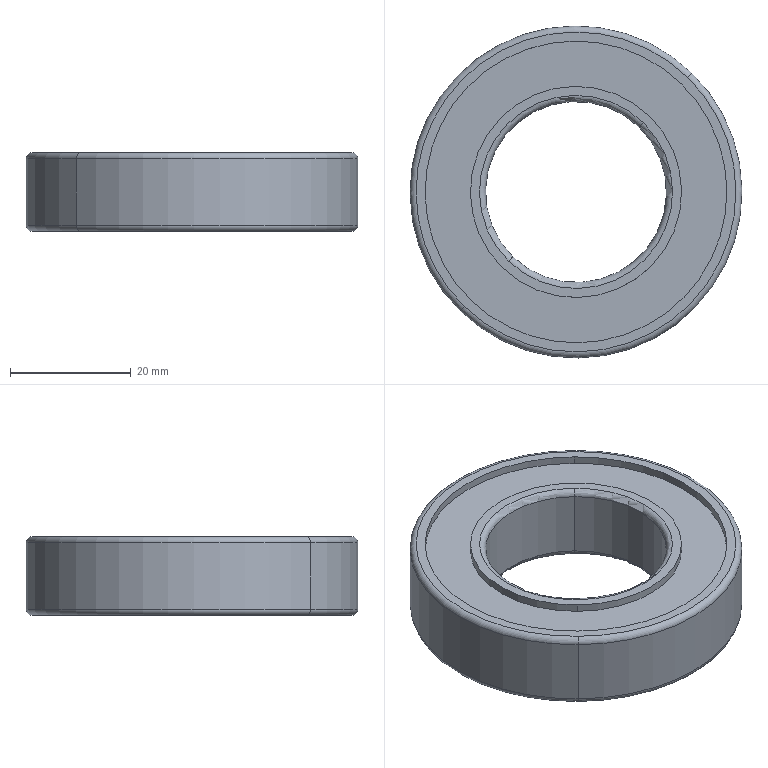Component | SolidWorks | 12AEncoderWheel-1_12A6006RZBearing-1 | 1 solid | 26 faces | box 55 x 55 x 13 mm | volume 18978 mm3 | cylinder 12 | torus 8 | plane 6 | commonest cylinder face diameters 50 x4 35 x4 55 x2 30 x2
STEP:
#1=CARTESIAN_POINT('',(5.515,6.57,0.2657));
#2=VERTEX_POINT('',#1);
#3=CARTESIAN_POINT('',(4.004,5.019,0.2657));
#4=VERTEX_POINT('',#3);
#5=CARTESIAN_POINT('',(4.76,5.795,0.2657));
#6=DIRECTION('',(0.,0.,1.));
#7=DIRECTION('',(-0.6982,-0.7159,0.));
#8=AXIS2_PLACEMENT_3D('',#5,#6,#7);
#9=CIRCLE('',#8,1.083);
#10=EDGE_CURVE('',#2,#4,#9,.T.);
#11=ORIENTED_EDGE('',*,*,#10,.F.);
#12=CARTESIAN_POINT('',(5.515,6.57,-0.1673));
#13=VERTEX_POINT('',#12);
#14=CARTESIAN_POINT('',(5.515,6.57,197.156));
#15=DIRECTION('',(-0.,-0.,-1.));
#16=VECTOR('',#15,39.37);
#17=LINE('',#14,#16);
#18=EDGE_CURVE('',#2,#13,#17,.T.);
#19=ORIENTED_EDGE('',*,*,#18,.T.);
#20=CARTESIAN_POINT('',(4.004,5.019,-0.1673));
#21=VERTEX_POINT('',#20);
#22=CARTESIAN_POINT('',(4.76,5.795,-0.1673));
#23=DIRECTION('',(0.,0.,1.));
#24=DIRECTION('',(-0.6982,-0.7159,0.));
#25=AXIS2_PLACEMENT_3D('',#22,#23,#24);
#26=CIRCLE('',#25,1.083);
#27=EDGE_CURVE('',#13,#21,#26,.T.);
#28=ORIENTED_EDGE('',*,*,#27,.T.);
#29=CARTESIAN_POINT('',(4.004,5.019,197.156));
#30=DIRECTION('',(-0.,-0.,-1.));
#31=VECTOR('',#30,39.37);
#32=LINE('',#29,#31);
#33=EDGE_CURVE('',#4,#21,#32,.T.);
#34=ORIENTED_EDGE('',*,*,#33,.F.);
#35=EDGE_LOOP('',(#11,#19,#28,#34));
#36=FACE_OUTER_BOUND('',#35,.T.);
#37=CARTESIAN_POINT('',(4.76,5.795,197.156));
#38=DIRECTION('',(-0.,-0.,-1.));
#39=DIRECTION('',(-0.6982,-0.7159,0.));
#40=AXIS2_PLACEMENT_3D('',#37,#38,#39);
#41=CYLINDRICAL_SURFACE('',#40,1.083);
#42=ADVANCED_FACE('',(#36),#41,.T.);
#43=CARTESIAN_POINT('',(4.76,5.795,0.2657));
#44=DIRECTION('',(0.,0.,1.));
#45=DIRECTION('',(-0.6982,-0.7159,0.));
#46=AXIS2_PLACEMENT_3D('',#43,#44,#45);
#47=CIRCLE('',#46,1.083);
#48=EDGE_CURVE('',#4,#2,#47,.T.);
#49=ORIENTED_EDGE('',*,*,#48,.T.);
#50=CARTESIAN_POINT('',(5.488,6.541,0.3051));
#51=VERTEX_POINT('',#50);
#52=CARTESIAN_POINT('',(5.488,6.541,0.2657));
#53=DIRECTION('',(0.7159,-0.6982,0.));
#54=DIRECTION('',(0.6982,0.7159,0.));
#55=AXIS2_PLACEMENT_3D('',#52,#53,#54);
#56=CIRCLE('',#55,0.03937);
#57=EDGE_CURVE('',#2,#51,#56,.T.);
#58=ORIENTED_EDGE('',*,*,#57,.T.);
#59=CARTESIAN_POINT('',(4.031,5.048,0.3051));
#60=VERTEX_POINT('',#59);
#61=CARTESIAN_POINT('',(4.76,5.795,0.3051));
#62=DIRECTION('',(0.,0.,1.));
#63=DIRECTION('',(-0.6982,-0.7159,0.));
#64=AXIS2_PLACEMENT_3D('',#61,#62,#63);
#65=CIRCLE('',#64,1.043);
#66=EDGE_CURVE('',#60,#51,#65,.T.);
#67=ORIENTED_EDGE('',*,*,#66,.F.);
#68=CARTESIAN_POINT('',(4.031,5.048,0.2657));
#69=DIRECTION('',(-0.7159,0.6982,-0.));
#70=DIRECTION('',(-0.6982,-0.7159,0.));
#71=AXIS2_PLACEMENT_3D('',#68,#69,#70);
#72=CIRCLE('',#71,0.03937);
#73=EDGE_CURVE('',#4,#60,#72,.T.);
#74=ORIENTED_EDGE('',*,*,#73,.F.);
#75=EDGE_LOOP('',(#49,#58,#67,#74));
#76=FACE_OUTER_BOUND('',#75,.T.);
#77=CARTESIAN_POINT('',(4.76,5.795,0.2657));
#78=DIRECTION('',(0.,0.,1.));
#79=DIRECTION('',(-0.6982,-0.7159,0.));
#80=AXIS2_PLACEMENT_3D('',#77,#78,#79);
#81=TOROIDAL_SURFACE('',#80,1.043,0.03937);
#82=ADVANCED_FACE('',(#76),#81,.T.);
#83=CARTESIAN_POINT('',(4.072,5.09,0.3051));
#84=VERTEX_POINT('',#83);
#85=CARTESIAN_POINT('',(5.447,6.499,0.3051));
#86=VERTEX_POINT('',#85);
#87=CARTESIAN_POINT('',(4.76,5.795,0.3051));
#88=DIRECTION('',(0.,0.,1.));
#89=DIRECTION('',(-0.6982,-0.7159,0.));
#90=AXIS2_PLACEMENT_3D('',#87,#88,#89);
#91=CIRCLE('',#90,0.9843);
#92=EDGE_CURVE('',#84,#86,#91,.T.);
#93=ORIENTED_EDGE('',*,*,#92,.T.);
#94=CARTESIAN_POINT('',(5.447,6.499,0.2539));
#95=VERTEX_POINT('',#94);
#96=CARTESIAN_POINT('',(5.447,6.499,197.156));
#97=DIRECTION('',(-0.,-0.,-1.));
#98=VECTOR('',#97,39.37);
#99=LINE('',#96,#98);
#100=EDGE_CURVE('',#86,#95,#99,.T.);
#101=ORIENTED_EDGE('',*,*,#100,.T.);
#102=CARTESIAN_POINT('',(4.072,5.09,0.2539));
#103=VERTEX_POINT('',#102);
#104=CARTESIAN_POINT('',(4.76,5.795,0.2539));
#105=DIRECTION('',(0.,0.,1.));
#106=DIRECTION('',(-0.6982,-0.7159,0.));
#107=AXIS2_PLACEMENT_3D('',#104,#105,#106);
#108=CIRCLE('',#107,0.9843);
#109=EDGE_CURVE('',#103,#95,#108,.T.);
#110=ORIENTED_EDGE('',*,*,#109,.F.);
#111=CARTESIAN_POINT('',(4.072,5.09,197.156));
#112=DIRECTION('',(-0.,-0.,-1.));
#113=VECTOR('',#112,39.37);
#114=LINE('',#111,#113);
#115=EDGE_CURVE('',#84,#103,#114,.T.);
#116=ORIENTED_EDGE('',*,*,#115,.F.);
#117=EDGE_LOOP('',(#93,#101,#110,#116));
#118=FACE_OUTER_BOUND('',#117,.T.);
#119=CARTESIAN_POINT('',(4.76,5.795,197.156));
#120=DIRECTION('',(-0.,-0.,-1.));
#121=DIRECTION('',(-0.6982,-0.7159,0.));
#122=AXIS2_PLACEMENT_3D('',#119,#120,#121);
#123=CYLINDRICAL_SURFACE('',#122,0.9843);
#124=ADVANCED_FACE('',(#118),#123,.F.);
#125=CARTESIAN_POINT('',(5.241,6.288,0.3051));
#126=VERTEX_POINT('',#125);
#127=CARTESIAN_POINT('',(4.279,5.301,0.3051));
#128=VERTEX_POINT('',#127);
#129=CARTESIAN_POINT('',(4.76,5.795,0.3051));
#130=DIRECTION('',(0.,0.,1.));
#131=DIRECTION('',(-0.6982,-0.7159,0.));
#132=AXIS2_PLACEMENT_3D('',#129,#130,#131);
#133=CIRCLE('',#132,0.689);
#134=EDGE_CURVE('',#126,#128,#133,.T.);
#135=ORIENTED_EDGE('',*,*,#134,.F.);
#136=CARTESIAN_POINT('',(5.241,6.288,0.2539));
#137=VERTEX_POINT('',#136);
#138=CARTESIAN_POINT('',(5.241,6.288,197.156));
#139=DIRECTION('',(-0.,-0.,-1.));
#140=VECTOR('',#139,39.37);
#141=LINE('',#138,#140);
#142=EDGE_CURVE('',#126,#137,#141,.T.);
#143=ORIENTED_EDGE('',*,*,#142,.T.);
#144=CARTESIAN_POINT('',(4.279,5.301,0.2539));
#145=VERTEX_POINT('',#144);
#146=CARTESIAN_POINT('',(4.76,5.795,0.2539));
#147=DIRECTION('',(0.,0.,1.));
#148=DIRECTION('',(-0.6982,-0.7159,0.));
#149=AXIS2_PLACEMENT_3D('',#146,#147,#148);
#150=CIRCLE('',#149,0.689);
#151=EDGE_CURVE('',#137,#145,#150,.T.);
#152=ORIENTED_EDGE('',*,*,#151,.T.);
#153=CARTESIAN_POINT('',(4.279,5.301,197.156));
#154=DIRECTION('',(-0.,-0.,-1.));
#155=VECTOR('',#154,39.37);
#156=LINE('',#153,#155);
#157=EDGE_CURVE('',#128,#145,#156,.T.);
#158=ORIENTED_EDGE('',*,*,#157,.F.);
#159=EDGE_LOOP('',(#135,#143,#152,#158));
#160=FACE_OUTER_BOUND('',#159,.T.);
#161=CARTESIAN_POINT('',(4.76,5.795,197.156));
#162=DIRECTION('',(-0.,-0.,-1.));
#163=DIRECTION('',(-0.6982,-0.7159,0.));
#164=AXIS2_PLACEMENT_3D('',#161,#162,#163);
#165=CYLINDRICAL_SURFACE('',#164,0.689);
#166=ADVANCED_FACE('',(#160),#165,.T.);
#167=CARTESIAN_POINT('',(4.32,5.344,0.3051));
#168=VERTEX_POINT('',#167);
#169=CARTESIAN_POINT('',(5.199,6.246,0.3051));
#170=VERTEX_POINT('',#169);
#171=CARTESIAN_POINT('',(4.76,5.795,0.3051));
#172=DIRECTION('',(0.,0.,1.));
#173=DIRECTION('',(-0.6982,-0.7159,0.));
#174=AXIS2_PLACEMENT_3D('',#171,#172,#173);
#175=CIRCLE('',#174,0.6299);
#176=EDGE_CURVE('',#168,#170,#175,.T.);
#177=ORIENTED_EDGE('',*,*,#176,.T.);
#178=CARTESIAN_POINT('',(5.172,6.217,0.2657));
#179=VERTEX_POINT('',#178);
#180=CARTESIAN_POINT('',(5.199,6.246,0.2657));
#181=DIRECTION('',(0.7159,-0.6982,0.));
#182=DIRECTION('',(0.6982,0.7159,0.));
#183=AXIS2_PLACEMENT_3D('',#180,#181,#182);
#184=CIRCLE('',#183,0.03937);
#185=EDGE_CURVE('',#170,#179,#184,.T.);
#186=ORIENTED_EDGE('',*,*,#185,.T.);
#187=CARTESIAN_POINT('',(4.347,5.372,0.2657));
#188=VERTEX_POINT('',#187);
#189=CARTESIAN_POINT('',(4.76,5.795,0.2657));
#190=DIRECTION('',(0.,0.,1.));
#191=DIRECTION('',(-0.6982,-0.7159,0.));
#192=AXIS2_PLACEMENT_3D('',#189,#190,#191);
#193=CIRCLE('',#192,0.5906);
#194=EDGE_CURVE('',#188,#179,#193,.T.);
#195=ORIENTED_EDGE('',*,*,#194,.F.);
#196=CARTESIAN_POINT('',(4.32,5.344,0.2657));
#197=DIRECTION('',(-0.7159,0.6982,-0.));
#198=DIRECTION('',(-0.6982,-0.7159,0.));
#199=AXIS2_PLACEMENT_3D('',#196,#197,#198);
#200=CIRCLE('',#199,0.03937);
#201=EDGE_CURVE('',#168,#188,#200,.T.);
#202=ORIENTED_EDGE('',*,*,#201,.F.);
#203=EDGE_LOOP('',(#177,#186,#195,#202));
#204=FACE_OUTER_BOUND('',#203,.T.);
#205=CARTESIAN_POINT('',(4.76,5.795,0.2657));
#206=DIRECTION('',(0.,0.,1.));
#207=DIRECTION('',(-0.6982,-0.7159,0.));
#208=AXIS2_PLACEMENT_3D('',#205,#206,#207);
#209=TOROIDAL_SURFACE('',#208,0.6299,0.03937);
#210=ADVANCED_FACE('',(#204),#209,.T.);
#211=ORIENTED_EDGE('',*,*,#194,.T.);
#212=CARTESIAN_POINT('',(5.172,6.217,-0.1673));
#213=VERTEX_POINT('',#212);
#214=CARTESIAN_POINT('',(5.172,6.217,197.156));
#215=DIRECTION('',(-0.,-0.,-1.));
#216=VECTOR('',#215,39.37);
#217=LINE('',#214,#216);
#218=EDGE_CURVE('',#179,#213,#217,.T.);
#219=ORIENTED_EDGE('',*,*,#218,.T.);
#220=CARTESIAN_POINT('',(4.347,5.372,-0.1673));
#221=VERTEX_POINT('',#220);
#222=CARTESIAN_POINT('',(4.76,5.795,-0.1673));
#223=DIRECTION('',(0.,0.,1.));
#224=DIRECTION('',(-0.6982,-0.7159,0.));
#225=AXIS2_PLACEMENT_3D('',#222,#223,#224);
#226=CIRCLE('',#225,0.5906);
#227=EDGE_CURVE('',#221,#213,#226,.T.);
#228=ORIENTED_EDGE('',*,*,#227,.F.);
#229=CARTESIAN_POINT('',(4.347,5.372,197.156));
#230=DIRECTION('',(-0.,-0.,-1.));
#231=VECTOR('',#230,39.37);
#232=LINE('',#229,#231);
#233=EDGE_CURVE('',#188,#221,#232,.T.);
#234=ORIENTED_EDGE('',*,*,#233,.F.);
#235=EDGE_LOOP('',(#211,#219,#228,#234));
#236=FACE_OUTER_BOUND('',#235,.T.);
#237=CARTESIAN_POINT('',(4.76,5.795,197.156));
#238=DIRECTION('',(-0.,-0.,-1.));
#239=DIRECTION('',(-0.6982,-0.7159,0.));
#240=AXIS2_PLACEMENT_3D('',#237,#238,#239);
#241=CYLINDRICAL_SURFACE('',#240,0.5906);
#242=ADVANCED_FACE('',(#236),#241,.F.);
#243=ORIENTED_EDGE('',*,*,#227,.T.);
#244=CARTESIAN_POINT('',(5.199,6.246,-0.2067));
#245=VERTEX_POINT('',#244);
#246=CARTESIAN_POINT('',(5.199,6.246,-0.1673));
#247=DIRECTION('',(0.7159,-0.6982,0.));
#248=DIRECTION('',(0.6982,0.7159,0.));
#249=AXIS2_PLACEMENT_3D('',#246,#247,#248);
#250=CIRCLE('',#249,0.03937);
#251=EDGE_CURVE('',#213,#245,#250,.T.);
#252=ORIENTED_EDGE('',*,*,#251,.T.);
#253=CARTESIAN_POINT('',(4.32,5.344,-0.2067));
#254=VERTEX_POINT('',#253);
#255=CARTESIAN_POINT('',(4.76,5.795,-0.2067));
#256=DIRECTION('',(0.,0.,1.));
#257=DIRECTION('',(-0.6982,-0.7159,0.));
#258=AXIS2_PLACEMENT_3D('',#255,#256,#257);
#259=CIRCLE('',#258,0.6299);
#260=EDGE_CURVE('',#254,#245,#259,.T.);
#261=ORIENTED_EDGE('',*,*,#260,.F.);
#262=CARTESIAN_POINT('',(4.32,5.344,-0.1673));
#263=DIRECTION('',(-0.7159,0.6982,-0.));
#264=DIRECTION('',(-0.6982,-0.7159,0.));
#265=AXIS2_PLACEMENT_3D('',#262,#263,#264);
#266=CIRCLE('',#265,0.03937);
#267=EDGE_CURVE('',#221,#254,#266,.T.);
#268=ORIENTED_EDGE('',*,*,#267,.F.);
#269=EDGE_LOOP('',(#243,#252,#261,#268));
#270=FACE_OUTER_BOUND('',#269,.T.);
#271=CARTESIAN_POINT('',(4.76,5.795,-0.1673));
#272=DIRECTION('',(0.,0.,1.));
#273=DIRECTION('',(-0.6982,-0.7159,0.));
#274=AXIS2_PLACEMENT_3D('',#271,#272,#273);
#275=TOROIDAL_SURFACE('',#274,0.6299,0.03937);
#276=ADVANCED_FACE('',(#270),#275,.T.);
#277=CARTESIAN_POINT('',(5.241,6.288,-0.1555));
#278=VERTEX_POINT('',#277);
#279=CARTESIAN_POINT('',(4.279,5.301,-0.1555));
#280=VERTEX_POINT('',#279);
#281=CARTESIAN_POINT('',(4.76,5.795,-0.1555));
#282=DIRECTION('',(0.,0.,1.));
#283=DIRECTION('',(-0.6982,-0.7159,0.));
#284=AXIS2_PLACEMENT_3D('',#281,#282,#283);
#285=CIRCLE('',#284,0.689);
#286=EDGE_CURVE('',#278,#280,#285,.T.);
#287=ORIENTED_EDGE('',*,*,#286,.F.);
#288=CARTESIAN_POINT('',(5.241,6.288,-0.2067));
#289=VERTEX_POINT('',#288);
#290=CARTESIAN_POINT('',(5.241,6.288,197.156));
#291=DIRECTION('',(-0.,-0.,-1.));
#292=VECTOR('',#291,39.37);
#293=LINE('',#290,#292);
#294=EDGE_CURVE('',#278,#289,#293,.T.);
#295=ORIENTED_EDGE('',*,*,#294,.T.);
#296=CARTESIAN_POINT('',(4.279,5.301,-0.2067));
#297=VERTEX_POINT('',#296);
#298=CARTESIAN_POINT('',(4.76,5.795,-0.2067));
#299=DIRECTION('',(0.,0.,1.));
#300=DIRECTION('',(-0.6982,-0.7159,0.));
#301=AXIS2_PLACEMENT_3D('',#298,#299,#300);
#302=CIRCLE('',#301,0.689);
#303=EDGE_CURVE('',#289,#297,#302,.T.);
#304=ORIENTED_EDGE('',*,*,#303,.T.);
#305=CARTESIAN_POINT('',(4.279,5.301,197.156));
#306=DIRECTION('',(-0.,-0.,-1.));
#307=VECTOR('',#306,39.37);
#308=LINE('',#305,#307);
#309=EDGE_CURVE('',#280,#297,#308,.T.);
#310=ORIENTED_EDGE('',*,*,#309,.F.);
#311=EDGE_LOOP('',(#287,#295,#304,#310));
#312=FACE_OUTER_BOUND('',#311,.T.);
#313=CARTESIAN_POINT('',(4.76,5.795,197.156));
#314=DIRECTION('',(-0.,-0.,-1.));
#315=DIRECTION('',(-0.6982,-0.7159,0.));
#316=AXIS2_PLACEMENT_3D('',#313,#314,#315);
#317=CYLINDRICAL_SURFACE('',#316,0.689);
#318=ADVANCED_FACE('',(#312),#317,.T.);
#319=CARTESIAN_POINT('',(4.072,5.09,-0.1555));
#320=VERTEX_POINT('',#319);
#321=CARTESIAN_POINT('',(5.447,6.499,-0.1555));
#322=VERTEX_POINT('',#321);
#323=CARTESIAN_POINT('',(4.76,5.795,-0.1555));
#324=DIRECTION('',(0.,0.,1.));
#325=DIRECTION('',(-0.6982,-0.7159,0.));
#326=AXIS2_PLACEMENT_3D('',#323,#324,#325);
#327=CIRCLE('',#326,0.9843);
#328=EDGE_CURVE('',#320,#322,#327,.T.);
#329=ORIENTED_EDGE('',*,*,#328,.T.);
#330=CARTESIAN_POINT('',(5.447,6.499,-0.2067));
#331=VERTEX_POINT('',#330);
#332=CARTESIAN_POINT('',(5.447,6.499,197.156));
#333=DIRECTION('',(-0.,-0.,-1.));
#334=VECTOR('',#333,39.37);
#335=LINE('',#332,#334);
#336=EDGE_CURVE('',#322,#331,#335,.T.);
#337=ORIENTED_EDGE('',*,*,#336,.T.);
#338=CARTESIAN_POINT('',(4.072,5.09,-0.2067));
#339=VERTEX_POINT('',#338);
#340=CARTESIAN_POINT('',(4.76,5.795,-0.2067));
#341=DIRECTION('',(0.,0.,1.));
#342=DIRECTION('',(-0.6982,-0.7159,0.));
#343=AXIS2_PLACEMENT_3D('',#340,#341,#342);
#344=CIRCLE('',#343,0.9843);
#345=EDGE_CURVE('',#339,#331,#344,.T.);
#346=ORIENTED_EDGE('',*,*,#345,.F.);
#347=CARTESIAN_POINT('',(4.072,5.09,197.156));
#348=DIRECTION('',(-0.,-0.,-1.));
#349=VECTOR('',#348,39.37);
#350=LINE('',#347,#349);
#351=EDGE_CURVE('',#320,#339,#350,.T.);
#352=ORIENTED_EDGE('',*,*,#351,.F.);
#353=EDGE_LOOP('',(#329,#337,#346,#352));
#354=FACE_OUTER_BOUND('',#353,.T.);
#355=CARTESIAN_POINT('',(4.76,5.795,197.156));
#356=DIRECTION('',(-0.,-0.,-1.));
#357=DIRECTION('',(-0.6982,-0.7159,0.));
#358=AXIS2_PLACEMENT_3D('',#355,#356,#357);
#359=CYLINDRICAL_SURFACE('',#358,0.9843);
#360=ADVANCED_FACE('',(#354),#359,.F.);
#361=CARTESIAN_POINT('',(4.031,5.048,-0.2067));
#362=VERTEX_POINT('',#361);
#363=CARTESIAN_POINT('',(5.488,6.541,-0.2067));
#364=VERTEX_POINT('',#363);
#365=CARTESIAN_POINT('',(4.76,5.795,-0.2067));
#366=DIRECTION('',(0.,0.,1.));
#367=DIRECTION('',(-0.6982,-0.7159,0.));
#368=AXIS2_PLACEMENT_3D('',#365,#366,#367);
#369=CIRCLE('',#368,1.043);
#370=EDGE_CURVE('',#362,#364,#369,.T.);
#371=ORIENTED_EDGE('',*,*,#370,.T.);
#372=CARTESIAN_POINT('',(5.488,6.541,-0.1673));
#373=DIRECTION('',(0.7159,-0.6982,0.));
#374=DIRECTION('',(0.6982,0.7159,0.));
#375=AXIS2_PLACEMENT_3D('',#372,#373,#374);
#376=CIRCLE('',#375,0.03937);
#377=EDGE_CURVE('',#364,#13,#376,.T.);
#378=ORIENTED_EDGE('',*,*,#377,.T.);
#379=CARTESIAN_POINT('',(4.76,5.795,-0.1673));
#380=DIRECTION('',(0.,0.,1.));
#381=DIRECTION('',(-0.6982,-0.7159,0.));
#382=AXIS2_PLACEMENT_3D('',#379,#380,#381);
#383=CIRCLE('',#382,1.083);
#384=EDGE_CURVE('',#21,#13,#383,.T.);
#385=ORIENTED_EDGE('',*,*,#384,.F.);
#386=CARTESIAN_POINT('',(4.031,5.048,-0.1673));
#387=DIRECTION('',(-0.7159,0.6982,-0.));
#388=DIRECTION('',(-0.6982,-0.7159,0.));
#389=AXIS2_PLACEMENT_3D('',#386,#387,#388);
#390=CIRCLE('',#389,0.03937);
#391=EDGE_CURVE('',#362,#21,#390,.T.);
#392=ORIENTED_EDGE('',*,*,#391,.F.);
#393=EDGE_LOOP('',(#371,#378,#385,#392));
#394=FACE_OUTER_BOUND('',#393,.T.);
#395=CARTESIAN_POINT('',(4.76,5.795,-0.1673));
#396=DIRECTION('',(0.,0.,1.));
#397=DIRECTION('',(-0.6982,-0.7159,0.));
#398=AXIS2_PLACEMENT_3D('',#395,#396,#397);
#399=TOROIDAL_SURFACE('',#398,1.043,0.03937);
#400=ADVANCED_FACE('',(#394),#399,.T.);
#401=ORIENTED_EDGE('',*,*,#377,.F.);
#402=CARTESIAN_POINT('',(4.76,5.795,-0.2067));
#403=DIRECTION('',(0.,0.,1.));
#404=DIRECTION('',(-0.6982,-0.7159,0.));
#405=AXIS2_PLACEMENT_3D('',#402,#403,#404);
#406=CIRCLE('',#405,1.043);
#407=EDGE_CURVE('',#364,#362,#406,.T.);
#408=ORIENTED_EDGE('',*,*,#407,.T.);
#409=ORIENTED_EDGE('',*,*,#391,.T.);
#410=ORIENTED_EDGE('',*,*,#27,.F.);
#411=EDGE_LOOP('',(#401,#408,#409,#410));
#412=FACE_OUTER_BOUND('',#411,.T.);
#413=CARTESIAN_POINT('',(4.76,5.795,-0.1673));
#414=DIRECTION('',(0.,0.,1.));
#415=DIRECTION('',(-0.6982,-0.7159,0.));
#416=AXIS2_PLACEMENT_3D('',#413,#414,#415);
#417=TOROIDAL_SURFACE('',#416,1.043,0.03937);
#418=ADVANCED_FACE('',(#412),#417,.T.);
#419=ORIENTED_EDGE('',*,*,#370,.F.);
#420=ORIENTED_EDGE('',*,*,#407,.F.);
#421=EDGE_LOOP('',(#419,#420));
#422=FACE_OUTER_BOUND('',#421,.T.);
#423=ORIENTED_EDGE('',*,*,#345,.T.);
#424=CARTESIAN_POINT('',(4.76,5.795,-0.2067));
#425=DIRECTION('',(0.,0.,1.));
#426=DIRECTION('',(-0.6982,-0.7159,0.));
#427=AXIS2_PLACEMENT_3D('',#424,#425,#426);
#428=CIRCLE('',#427,0.9843);
#429=EDGE_CURVE('',#331,#339,#428,.T.);
#430=ORIENTED_EDGE('',*,*,#429,.T.);
#431=EDGE_LOOP('',(#423,#430));
#432=FACE_BOUND('',#431,.T.);
#433=CARTESIAN_POINT('',(5.507,5.066,-0.2067));
#434=DIRECTION('',(-0.,-0.,-1.));
#435=DIRECTION('',(0.6982,0.7159,-0.));
#436=AXIS2_PLACEMENT_3D('',#433,#434,#435);
#437=PLANE('',#436);
#438=ADVANCED_FACE('',(#422,#432),#437,.T.);
#439=ORIENTED_EDGE('',*,*,#336,.F.);
#440=CARTESIAN_POINT('',(4.76,5.795,-0.1555));
#441=DIRECTION('',(0.,0.,1.));
#442=DIRECTION('',(-0.6982,-0.7159,0.));
#443=AXIS2_PLACEMENT_3D('',#440,#441,#442);
#444=CIRCLE('',#443,0.9843);
#445=EDGE_CURVE('',#322,#320,#444,.T.);
#446=ORIENTED_EDGE('',*,*,#445,.T.);
#447=ORIENTED_EDGE('',*,*,#351,.T.);
#448=ORIENTED_EDGE('',*,*,#429,.F.);
#449=EDGE_LOOP('',(#439,#446,#447,#448));
#450=FACE_OUTER_BOUND('',#449,.T.);
#451=CARTESIAN_POINT('',(4.76,5.795,197.156));
#452=DIRECTION('',(-0.,-0.,-1.));
#453=DIRECTION('',(-0.6982,-0.7159,0.));
#454=AXIS2_PLACEMENT_3D('',#451,#452,#453);
#455=CYLINDRICAL_SURFACE('',#454,0.9843);
#456=ADVANCED_FACE('',(#450),#455,.F.);
#457=ORIENTED_EDGE('',*,*,#328,.F.);
#458=ORIENTED_EDGE('',*,*,#445,.F.);
#459=EDGE_LOOP('',(#457,#458));
#460=FACE_OUTER_BOUND('',#459,.T.);
#461=CARTESIAN_POINT('',(4.76,5.795,-0.1555));
#462=DIRECTION('',(0.,0.,1.));
#463=DIRECTION('',(-0.6982,-0.7159,0.));
#464=AXIS2_PLACEMENT_3D('',#461,#462,#463);
#465=CIRCLE('',#464,0.689);
#466=EDGE_CURVE('',#280,#278,#465,.T.);
#467=ORIENTED_EDGE('',*,*,#466,.T.);
#468=ORIENTED_EDGE('',*,*,#286,.T.);
#469=EDGE_LOOP('',(#467,#468));
#470=FACE_BOUND('',#469,.T.);
#471=CARTESIAN_POINT('',(5.464,5.107,-0.1555));
#472=DIRECTION('',(-0.,-0.,-1.));
#473=DIRECTION('',(0.6982,0.7159,-0.));
#474=AXIS2_PLACEMENT_3D('',#471,#472,#473);
#475=PLANE('',#474);
#476=ADVANCED_FACE('',(#460,#470),#475,.T.);
#477=ORIENTED_EDGE('',*,*,#294,.F.);
#478=ORIENTED_EDGE('',*,*,#466,.F.);
#479=ORIENTED_EDGE('',*,*,#309,.T.);
#480=CARTESIAN_POINT('',(4.76,5.795,-0.2067));
#481=DIRECTION('',(0.,0.,1.));
#482=DIRECTION('',(-0.6982,-0.7159,0.));
#483=AXIS2_PLACEMENT_3D('',#480,#481,#482);
#484=CIRCLE('',#483,0.689);
#485=EDGE_CURVE('',#297,#289,#484,.T.);
#486=ORIENTED_EDGE('',*,*,#485,.T.);
#487=EDGE_LOOP('',(#477,#478,#479,#486));
#488=FACE_OUTER_BOUND('',#487,.T.);
#489=CARTESIAN_POINT('',(4.76,5.795,197.156));
#490=DIRECTION('',(-0.,-0.,-1.));
#491=DIRECTION('',(-0.6982,-0.7159,0.));
#492=AXIS2_PLACEMENT_3D('',#489,#490,#491);
#493=CYLINDRICAL_SURFACE('',#492,0.689);
#494=ADVANCED_FACE('',(#488),#493,.T.);
#495=ORIENTED_EDGE('',*,*,#485,.F.);
#496=ORIENTED_EDGE('',*,*,#303,.F.);
#497=EDGE_LOOP('',(#495,#496));
#498=FACE_OUTER_BOUND('',#497,.T.);
#499=ORIENTED_EDGE('',*,*,#260,.T.);
#500=CARTESIAN_POINT('',(4.76,5.795,-0.2067));
#501=DIRECTION('',(0.,0.,1.));
#502=DIRECTION('',(-0.6982,-0.7159,0.));
#503=AXIS2_PLACEMENT_3D('',#500,#501,#502);
#504=CIRCLE('',#503,0.6299);
#505=EDGE_CURVE('',#245,#254,#504,.T.);
#506=ORIENTED_EDGE('',*,*,#505,.T.);
#507=EDGE_LOOP('',(#499,#506));
#508=FACE_BOUND('',#507,.T.);
#509=CARTESIAN_POINT('',(5.253,5.314,-0.2067));
#510=DIRECTION('',(-0.,-0.,-1.));
#511=DIRECTION('',(0.6982,0.7159,-0.));
#512=AXIS2_PLACEMENT_3D('',#509,#510,#511);
#513=PLANE('',#512);
#514=ADVANCED_FACE('',(#498,#508),#513,.T.);
#515=ORIENTED_EDGE('',*,*,#251,.F.);
#516=CARTESIAN_POINT('',(4.76,5.795,-0.1673));
#517=DIRECTION('',(0.,0.,1.));
#518=DIRECTION('',(-0.6982,-0.7159,0.));
#519=AXIS2_PLACEMENT_3D('',#516,#517,#518);
#520=CIRCLE('',#519,0.5906);
#521=EDGE_CURVE('',#213,#221,#520,.T.);
#522=ORIENTED_EDGE('',*,*,#521,.T.);
#523=ORIENTED_EDGE('',*,*,#267,.T.);
#524=ORIENTED_EDGE('',*,*,#505,.F.);
#525=EDGE_LOOP('',(#515,#522,#523,#524));
#526=FACE_OUTER_BOUND('',#525,.T.);
#527=CARTESIAN_POINT('',(4.76,5.795,-0.1673));
#528=DIRECTION('',(0.,0.,1.));
#529=DIRECTION('',(-0.6982,-0.7159,0.));
#530=AXIS2_PLACEMENT_3D('',#527,#528,#529);
#531=TOROIDAL_SURFACE('',#530,0.6299,0.03937);
#532=ADVANCED_FACE('',(#526),#531,.T.);
#533=ORIENTED_EDGE('',*,*,#218,.F.);
#534=CARTESIAN_POINT('',(4.76,5.795,0.2657));
#535=DIRECTION('',(0.,0.,1.));
#536=DIRECTION('',(-0.6982,-0.7159,0.));
#537=AXIS2_PLACEMENT_3D('',#534,#535,#536);
#538=CIRCLE('',#537,0.5906);
#539=EDGE_CURVE('',#179,#188,#538,.T.);
#540=ORIENTED_EDGE('',*,*,#539,.T.);
#541=ORIENTED_EDGE('',*,*,#233,.T.);
#542=ORIENTED_EDGE('',*,*,#521,.F.);
#543=EDGE_LOOP('',(#533,#540,#541,#542));
#544=FACE_OUTER_BOUND('',#543,.T.);
#545=CARTESIAN_POINT('',(4.76,5.795,197.156));
#546=DIRECTION('',(-0.,-0.,-1.));
#547=DIRECTION('',(-0.6982,-0.7159,0.));
#548=AXIS2_PLACEMENT_3D('',#545,#546,#547);
#549=CYLINDRICAL_SURFACE('',#548,0.5906);
#550=ADVANCED_FACE('',(#544),#549,.F.);
#551=ORIENTED_EDGE('',*,*,#185,.F.);
#552=CARTESIAN_POINT('',(4.76,5.795,0.3051));
#553=DIRECTION('',(0.,0.,1.));
#554=DIRECTION('',(-0.6982,-0.7159,0.));
#555=AXIS2_PLACEMENT_3D('',#552,#553,#554);
#556=CIRCLE('',#555,0.6299);
#557=EDGE_CURVE('',#170,#168,#556,.T.);
#558=ORIENTED_EDGE('',*,*,#557,.T.);
#559=ORIENTED_EDGE('',*,*,#201,.T.);
#560=ORIENTED_EDGE('',*,*,#539,.F.);
#561=EDGE_LOOP('',(#551,#558,#559,#560));
#562=FACE_OUTER_BOUND('',#561,.T.);
#563=CARTESIAN_POINT('',(4.76,5.795,0.2657));
#564=DIRECTION('',(0.,0.,1.));
#565=DIRECTION('',(-0.6982,-0.7159,0.));
#566=AXIS2_PLACEMENT_3D('',#563,#564,#565);
#567=TOROIDAL_SURFACE('',#566,0.6299,0.03937);
#568=ADVANCED_FACE('',(#562),#567,.T.);
#569=CARTESIAN_POINT('',(4.76,5.795,0.3051));
#570=DIRECTION('',(0.,0.,1.));
#571=DIRECTION('',(-0.6982,-0.7159,0.));
#572=AXIS2_PLACEMENT_3D('',#569,#570,#571);
#573=CIRCLE('',#572,0.689);
#574=EDGE_CURVE('',#128,#126,#573,.T.);
#575=ORIENTED_EDGE('',*,*,#574,.T.);
#576=ORIENTED_EDGE('',*,*,#134,.T.);
#577=EDGE_LOOP('',(#575,#576));
#578=FACE_OUTER_BOUND('',#577,.T.);
#579=ORIENTED_EDGE('',*,*,#176,.F.);
#580=ORIENTED_EDGE('',*,*,#557,.F.);
#581=EDGE_LOOP('',(#579,#580));
#582=FACE_BOUND('',#581,.T.);
#583=CARTESIAN_POINT('',(5.211,5.355,0.3051));
#584=DIRECTION('',(0.,0.,1.));
#585=DIRECTION('',(0.7159,-0.6982,0.));
#586=AXIS2_PLACEMENT_3D('',#583,#584,#585);
#587=PLANE('',#586);
#588=ADVANCED_FACE('',(#578,#582),#587,.T.);
#589=ORIENTED_EDGE('',*,*,#142,.F.);
#590=ORIENTED_EDGE('',*,*,#574,.F.);
#591=ORIENTED_EDGE('',*,*,#157,.T.);
#592=CARTESIAN_POINT('',(4.76,5.795,0.2539));
#593=DIRECTION('',(0.,0.,1.));
#594=DIRECTION('',(-0.6982,-0.7159,0.));
#595=AXIS2_PLACEMENT_3D('',#592,#593,#594);
#596=CIRCLE('',#595,0.689);
#597=EDGE_CURVE('',#145,#137,#596,.T.);
#598=ORIENTED_EDGE('',*,*,#597,.T.);
#599=EDGE_LOOP('',(#589,#590,#591,#598));
#600=FACE_OUTER_BOUND('',#599,.T.);
#601=CARTESIAN_POINT('',(4.76,5.795,197.156));
#602=DIRECTION('',(-0.,-0.,-1.));
#603=DIRECTION('',(-0.6982,-0.7159,0.));
#604=AXIS2_PLACEMENT_3D('',#601,#602,#603);
#605=CYLINDRICAL_SURFACE('',#604,0.689);
#606=ADVANCED_FACE('',(#600),#605,.T.);
#607=ORIENTED_EDGE('',*,*,#109,.T.);
#608=CARTESIAN_POINT('',(4.76,5.795,0.2539));
#609=DIRECTION('',(0.,0.,1.));
#610=DIRECTION('',(-0.6982,-0.7159,0.));
#611=AXIS2_PLACEMENT_3D('',#608,#609,#610);
#612=CIRCLE('',#611,0.9843);
#613=EDGE_CURVE('',#95,#103,#612,.T.);
#614=ORIENTED_EDGE('',*,*,#613,.T.);
#615=EDGE_LOOP('',(#607,#614));
#616=FACE_OUTER_BOUND('',#615,.T.);
#617=ORIENTED_EDGE('',*,*,#597,.F.);
#618=ORIENTED_EDGE('',*,*,#151,.F.);
#619=EDGE_LOOP('',(#617,#618));
#620=FACE_BOUND('',#619,.T.);
#621=CARTESIAN_POINT('',(5.253,5.314,0.2539));
#622=DIRECTION('',(0.,0.,1.));
#623=DIRECTION('',(0.7159,-0.6982,0.));
#624=AXIS2_PLACEMENT_3D('',#621,#622,#623);
#625=PLANE('',#624);
#626=ADVANCED_FACE('',(#616,#620),#625,.T.);
#627=ORIENTED_EDGE('',*,*,#100,.F.);
#628=CARTESIAN_POINT('',(4.76,5.795,0.3051));
#629=DIRECTION('',(0.,0.,1.));
#630=DIRECTION('',(-0.6982,-0.7159,0.));
#631=AXIS2_PLACEMENT_3D('',#628,#629,#630);
#632=CIRCLE('',#631,0.9843);
#633=EDGE_CURVE('',#86,#84,#632,.T.);
#634=ORIENTED_EDGE('',*,*,#633,.T.);
#635=ORIENTED_EDGE('',*,*,#115,.T.);
#636=ORIENTED_EDGE('',*,*,#613,.F.);
#637=EDGE_LOOP('',(#627,#634,#635,#636));
#638=FACE_OUTER_BOUND('',#637,.T.);
#639=CARTESIAN_POINT('',(4.76,5.795,197.156));
#640=DIRECTION('',(-0.,-0.,-1.));
#641=DIRECTION('',(-0.6982,-0.7159,0.));
#642=AXIS2_PLACEMENT_3D('',#639,#640,#641);
#643=CYLINDRICAL_SURFACE('',#642,0.9843);
#644=ADVANCED_FACE('',(#638),#643,.F.);
#645=ORIENTED_EDGE('',*,*,#66,.T.);
#646=CARTESIAN_POINT('',(4.76,5.795,0.3051));
#647=DIRECTION('',(0.,0.,1.));
#648=DIRECTION('',(-0.6982,-0.7159,0.));
#649=AXIS2_PLACEMENT_3D('',#646,#647,#648);
#650=CIRCLE('',#649,1.043);
#651=EDGE_CURVE('',#51,#60,#650,.T.);
#652=ORIENTED_EDGE('',*,*,#651,.T.);
#653=EDGE_LOOP('',(#645,#652));
#654=FACE_OUTER_BOUND('',#653,.T.);
#655=ORIENTED_EDGE('',*,*,#92,.F.);
#656=ORIENTED_EDGE('',*,*,#633,.F.);
#657=EDGE_LOOP('',(#655,#656));
#658=FACE_BOUND('',#657,.T.);
#659=CARTESIAN_POINT('',(5.464,5.107,0.3051));
#660=DIRECTION('',(0.,0.,1.));
#661=DIRECTION('',(0.7159,-0.6982,0.));
#662=AXIS2_PLACEMENT_3D('',#659,#660,#661);
#663=PLANE('',#662);
#664=ADVANCED_FACE('',(#654,#658),#663,.T.);
#665=ORIENTED_EDGE('',*,*,#57,.F.);
#666=ORIENTED_EDGE('',*,*,#10,.T.);
#667=ORIENTED_EDGE('',*,*,#73,.T.);
#668=ORIENTED_EDGE('',*,*,#651,.F.);
#669=EDGE_LOOP('',(#665,#666,#667,#668));
#670=FACE_OUTER_BOUND('',#669,.T.);
#671=CARTESIAN_POINT('',(4.76,5.795,0.2657));
#672=DIRECTION('',(0.,0.,1.));
#673=DIRECTION('',(-0.6982,-0.7159,0.));
#674=AXIS2_PLACEMENT_3D('',#671,#672,#673);
#675=TOROIDAL_SURFACE('',#674,1.043,0.03937);
#676=ADVANCED_FACE('',(#670),#675,.T.);
#677=ORIENTED_EDGE('',*,*,#18,.F.);
#678=ORIENTED_EDGE('',*,*,#48,.F.);
#679=ORIENTED_EDGE('',*,*,#33,.T.);
#680=ORIENTED_EDGE('',*,*,#384,.T.);
#681=EDGE_LOOP('',(#677,#678,#679,#680));
#682=FACE_OUTER_BOUND('',#681,.T.);
#683=CARTESIAN_POINT('',(4.76,5.795,197.156));
#684=DIRECTION('',(-0.,-0.,-1.));
#685=DIRECTION('',(-0.6982,-0.7159,0.));
#686=AXIS2_PLACEMENT_3D('',#683,#684,#685);
#687=CYLINDRICAL_SURFACE('',#686,1.083);
#688=ADVANCED_FACE('',(#682),#687,.T.);
#689=CLOSED_SHELL('',(#42,#82,#124,#166,#210,#242,#276,#318,#360,#400,#418,#438,#456,#476,#494,#514,#532,#550,#568,#588,#606,#626,#644,#664,#676,#688));
#690=MANIFOLD_SOLID_BREP('',#689);
#691=CARTESIAN_POINT('',(0.,0.,0.));
#692=DIRECTION('',(0.,0.,1.));
#693=DIRECTION('',(1.,0.,0.));
#694=AXIS2_PLACEMENT_3D('',#691,#692,#693);
#695=(LENGTH_UNIT()NAMED_UNIT(*)SI_UNIT($,.METRE.));
#696=LENGTH_MEASURE_WITH_UNIT(LENGTH_MEASURE(0.0254),#695);
#697=DIMENSIONAL_EXPONENTS(1.,0.,0.,0.,0.,0.,0.);
#698=(CONVERSION_BASED_UNIT('',#696)LENGTH_UNIT()NAMED_UNIT(#697));
#699=UNCERTAINTY_MEASURE_WITH_UNIT(LENGTH_MEASURE(0.00001),#698,'','');
#700=(NAMED_UNIT(*)PLANE_ANGLE_UNIT()SI_UNIT($,.RADIAN.));
#701=(NAMED_UNIT(*)SI_UNIT($,.STERADIAN.)SOLID_ANGLE_UNIT());
#702=(GEOMETRIC_REPRESENTATION_CONTEXT(3)GLOBAL_UNCERTAINTY_ASSIGNED_CONTEXT((#699))GLOBAL_UNIT_ASSIGNED_CONTEXT((#698,#700,#701))REPRESENTATION_CONTEXT('',''));
#703=ADVANCED_BREP_SHAPE_REPRESENTATION('',(#690,#694),#702);
#704=COLOUR_RGB('',0.7922,0.8196,0.9333);
#705=FILL_AREA_STYLE_COLOUR('',#704);
#706=FILL_AREA_STYLE('',(#705));
#707=SURFACE_STYLE_FILL_AREA(#706);
#708=SURFACE_SIDE_STYLE('',(#707));
#709=SURFACE_STYLE_USAGE(.BOTH.,#708);
#710=PRESENTATION_STYLE_ASSIGNMENT((#709));
#711=STYLED_ITEM('',(#710),#690);
#712=(LENGTH_UNIT()NAMED_UNIT(*)SI_UNIT($,.METRE.));
#713=LENGTH_MEASURE_WITH_UNIT(LENGTH_MEASURE(0.0254),#712);
#714=DIMENSIONAL_EXPONENTS(1.,0.,0.,0.,0.,0.,0.);
#715=(CONVERSION_BASED_UNIT('',#713)LENGTH_UNIT()NAMED_UNIT(#714));
#716=UNCERTAINTY_MEASURE_WITH_UNIT(LENGTH_MEASURE(0.00001),#715,'','');
#717=(NAMED_UNIT(*)PLANE_ANGLE_UNIT()SI_UNIT($,.RADIAN.));
#718=(NAMED_UNIT(*)SI_UNIT($,.STERADIAN.)SOLID_ANGLE_UNIT());
#719=(GEOMETRIC_REPRESENTATION_CONTEXT(3)GLOBAL_UNCERTAINTY_ASSIGNED_CONTEXT((#716))GLOBAL_UNIT_ASSIGNED_CONTEXT((#715,#717,#718))REPRESENTATION_CONTEXT('',''));
#720=MECHANICAL_DESIGN_GEOMETRIC_PRESENTATION_REPRESENTATION('',(#711),#719);
#721=PRESENTATION_LAYER_ASSIGNMENT('','',(#711));